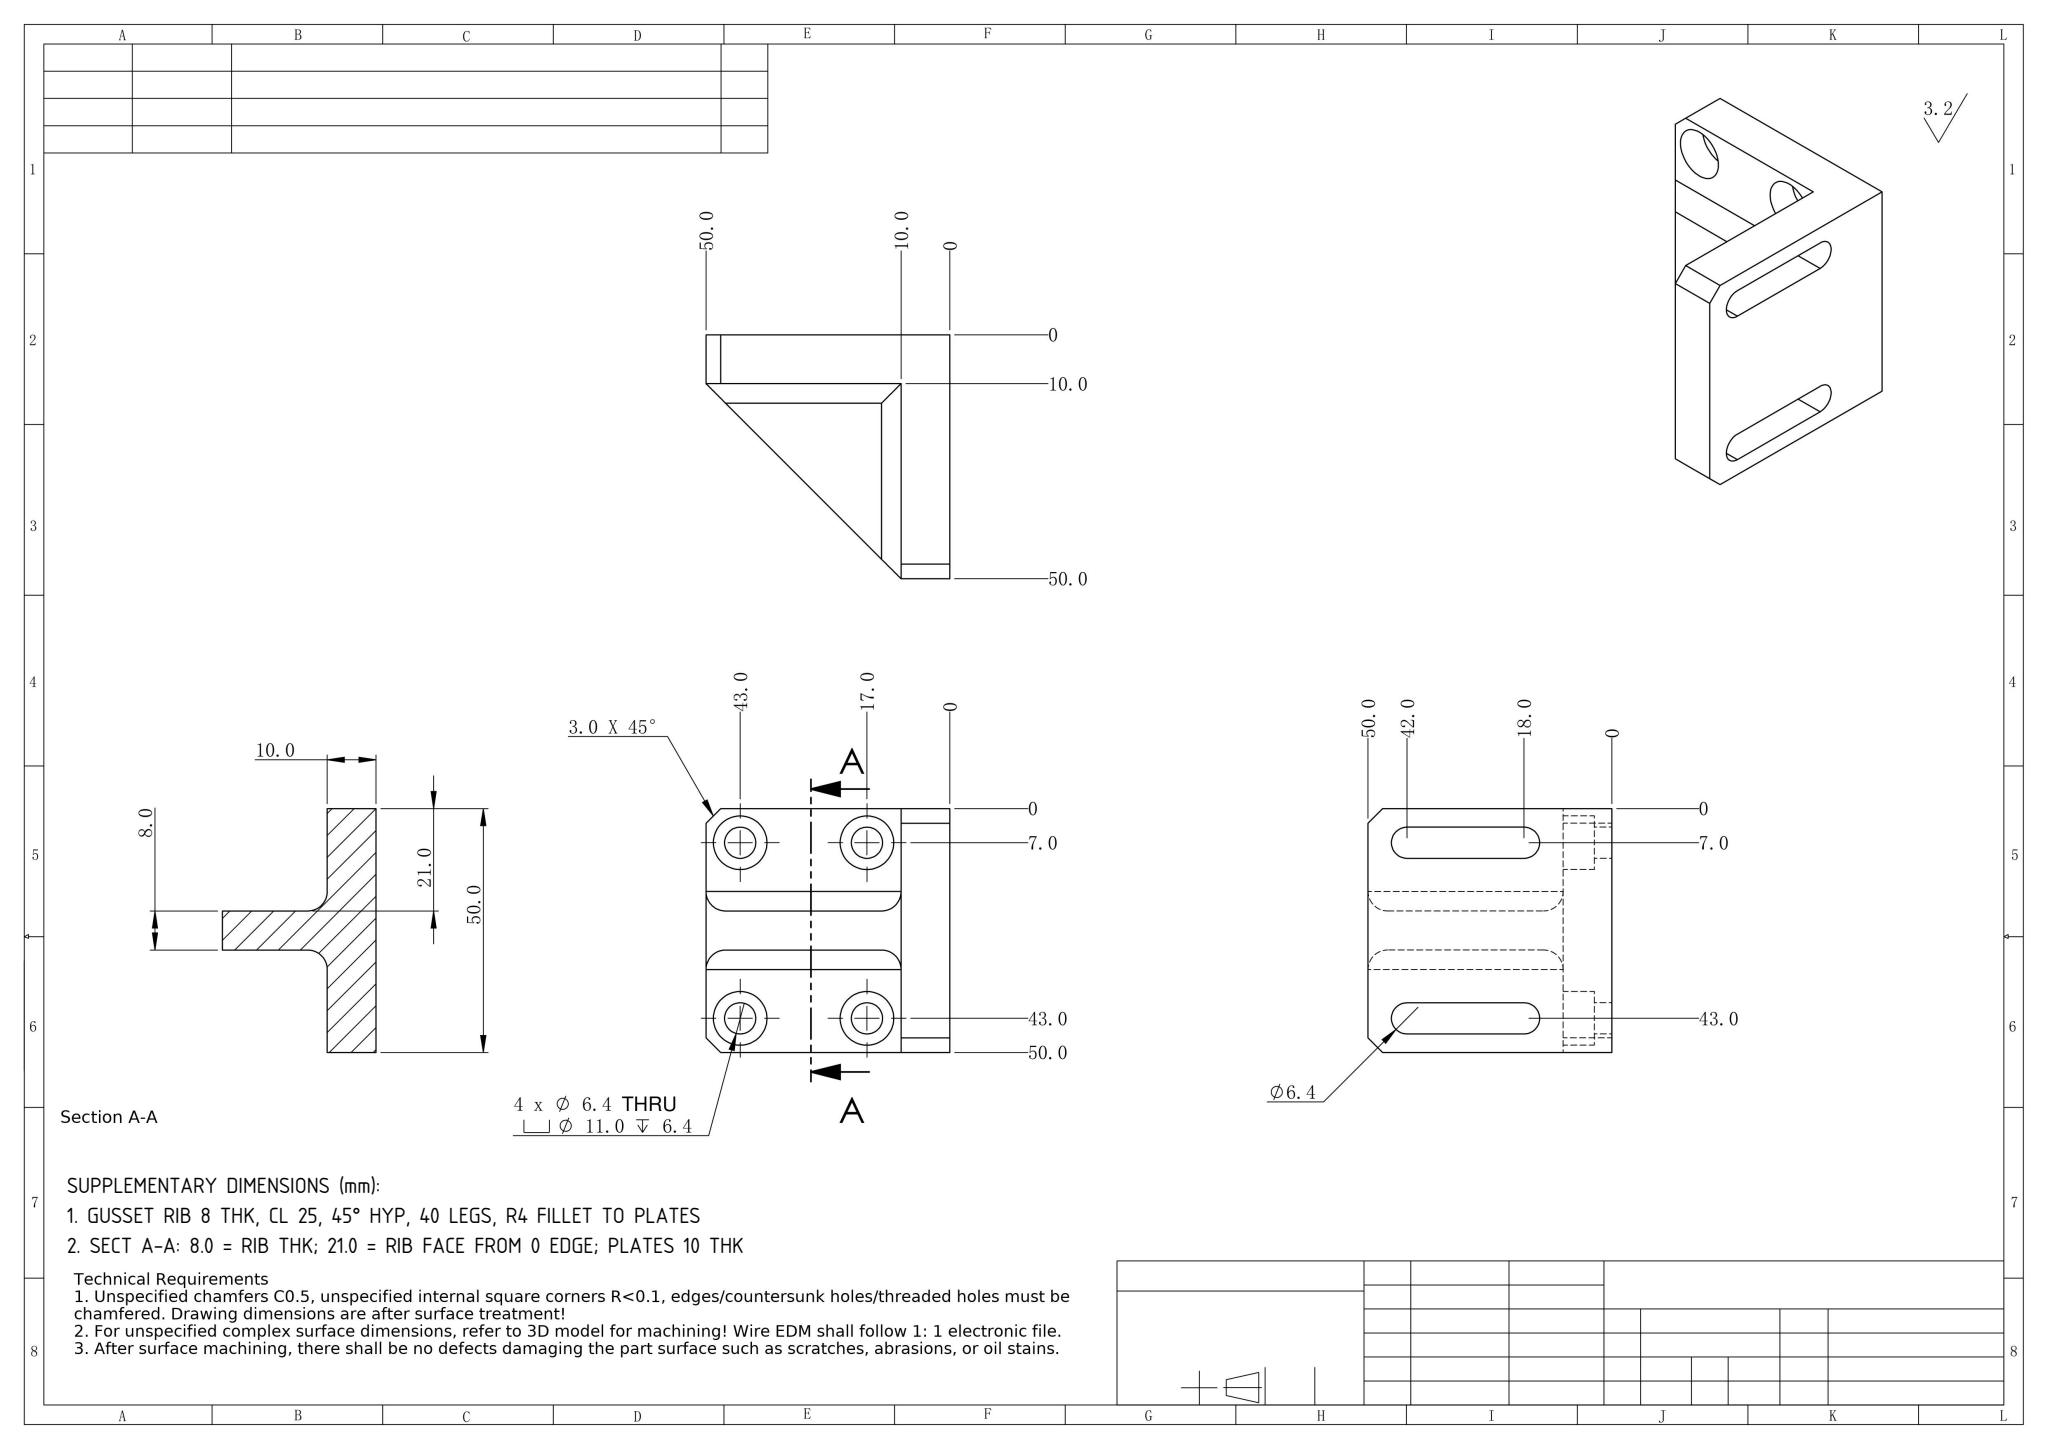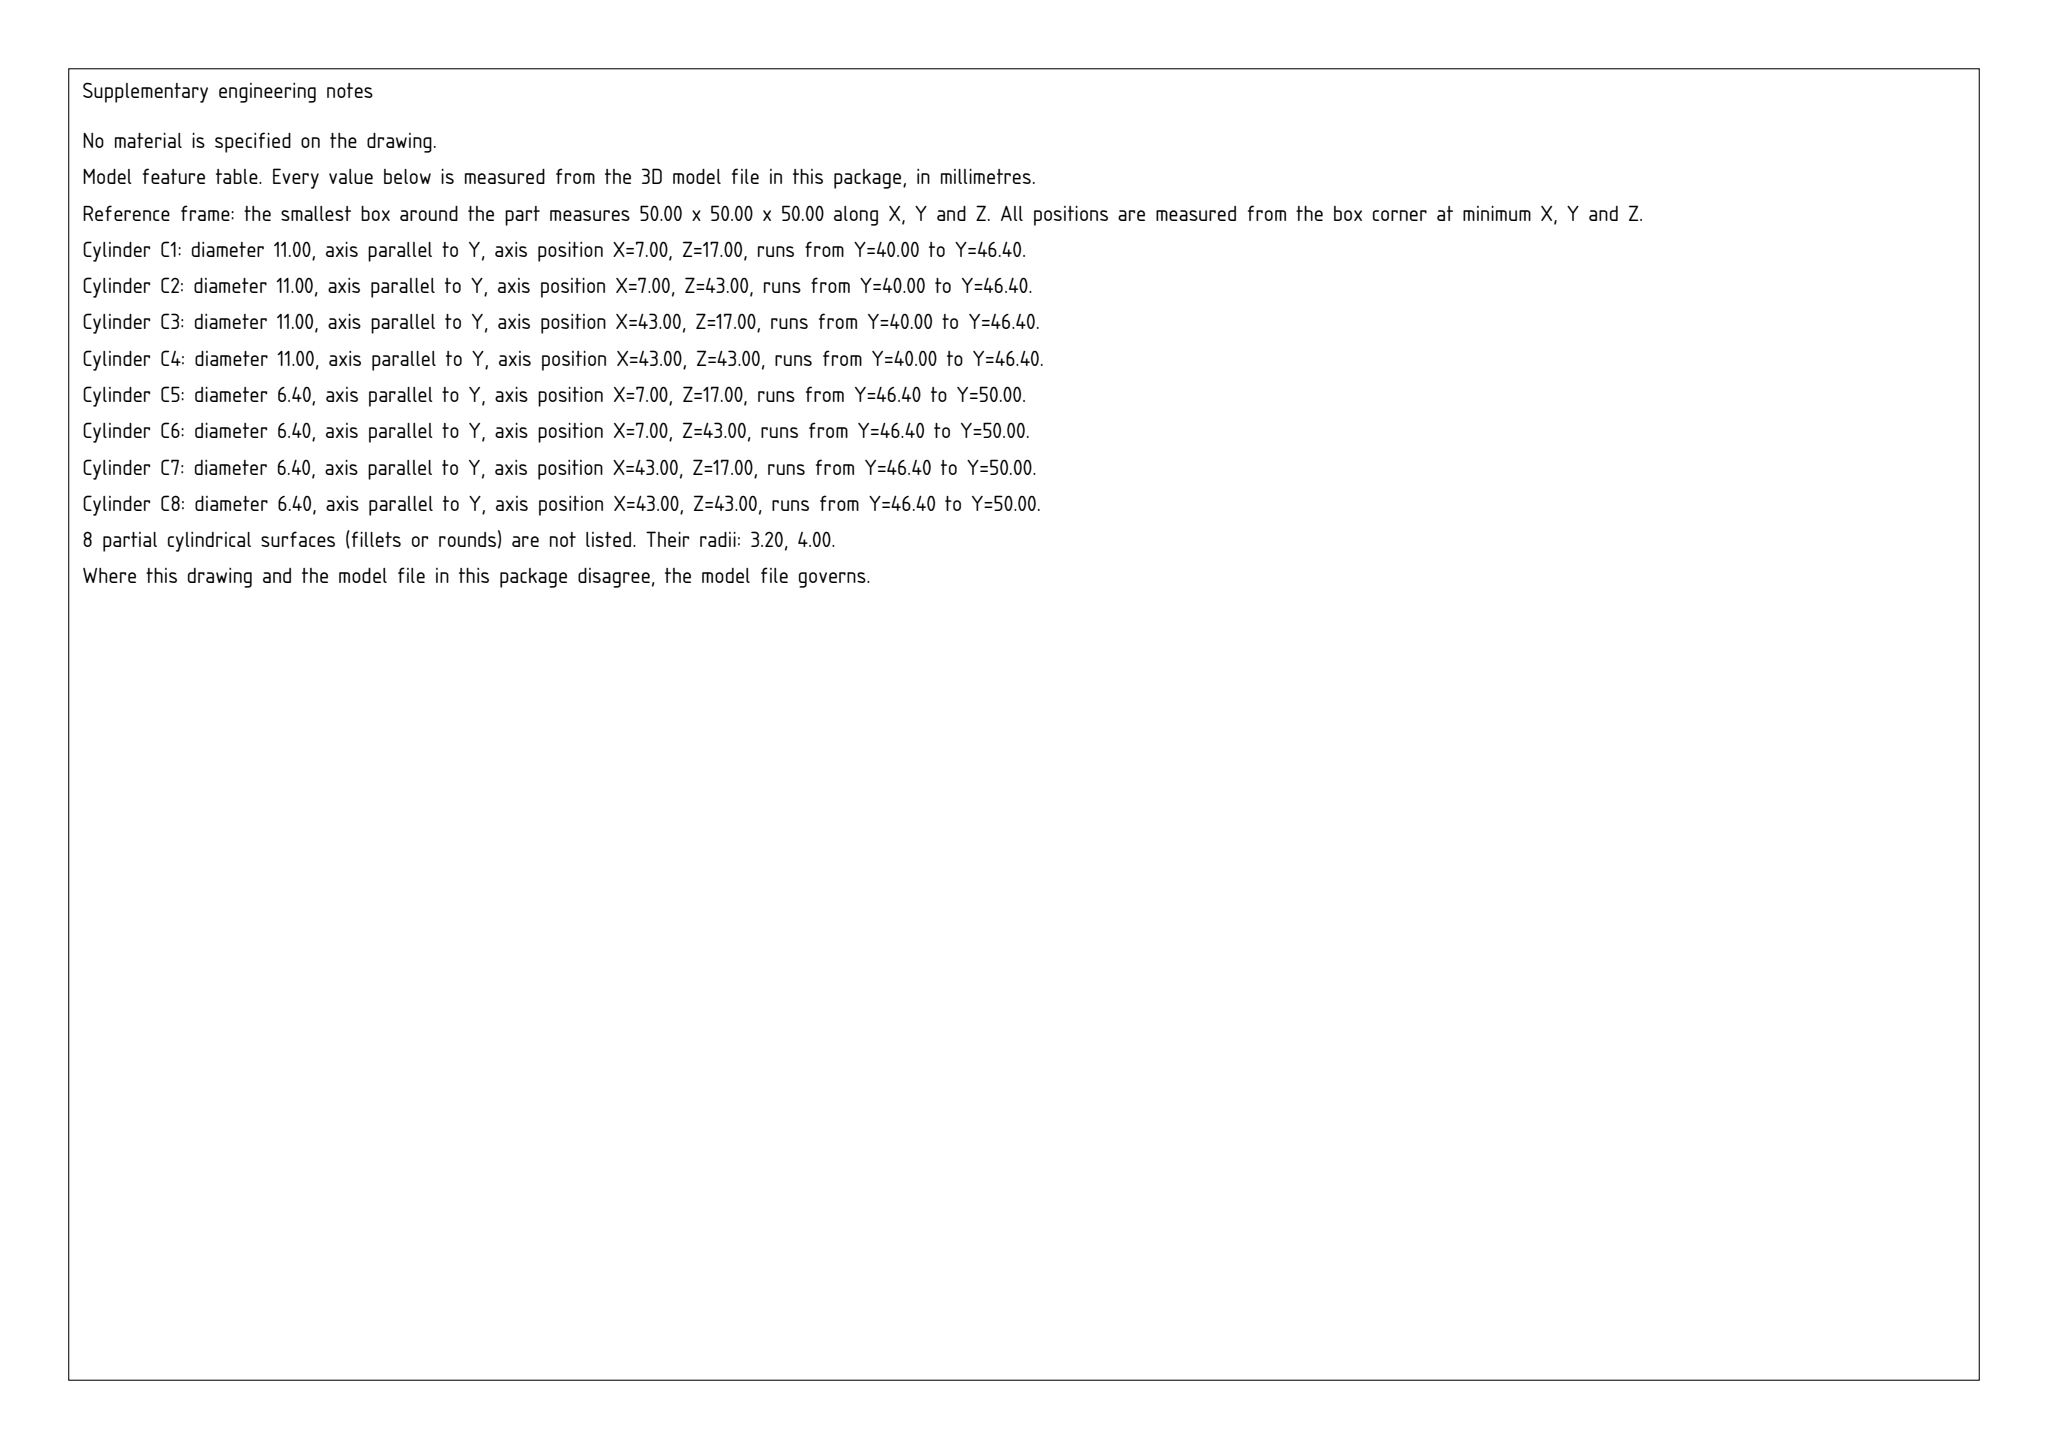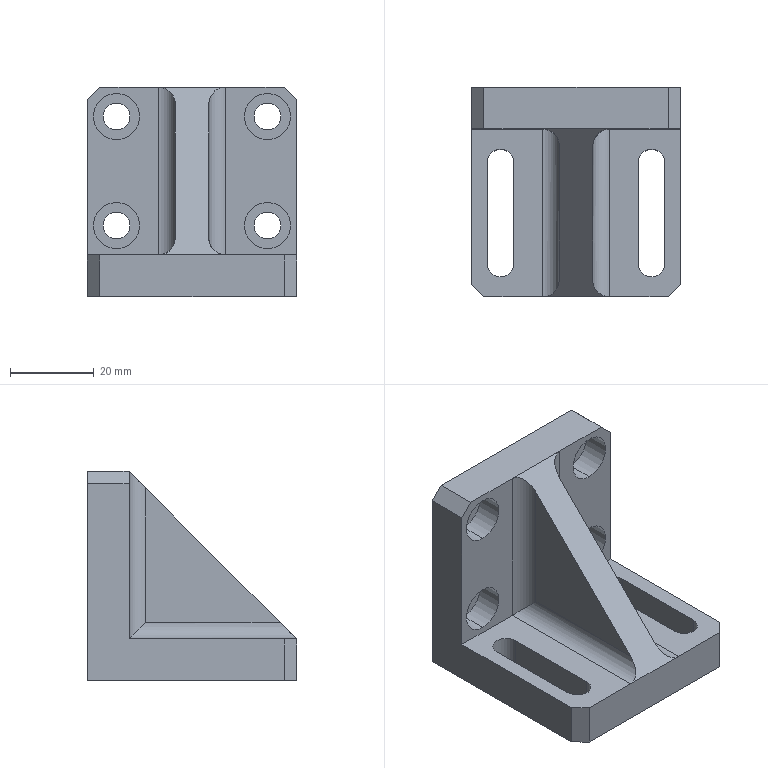Part | SolidWorks | mm | 1 solid | 49 faces | box 50 x 50 x 50 mm | volume 45133 mm3 | plane 25 | cylinder 24 | commonest cylinder face diameters 6.4 x12 11 x8 8 x4